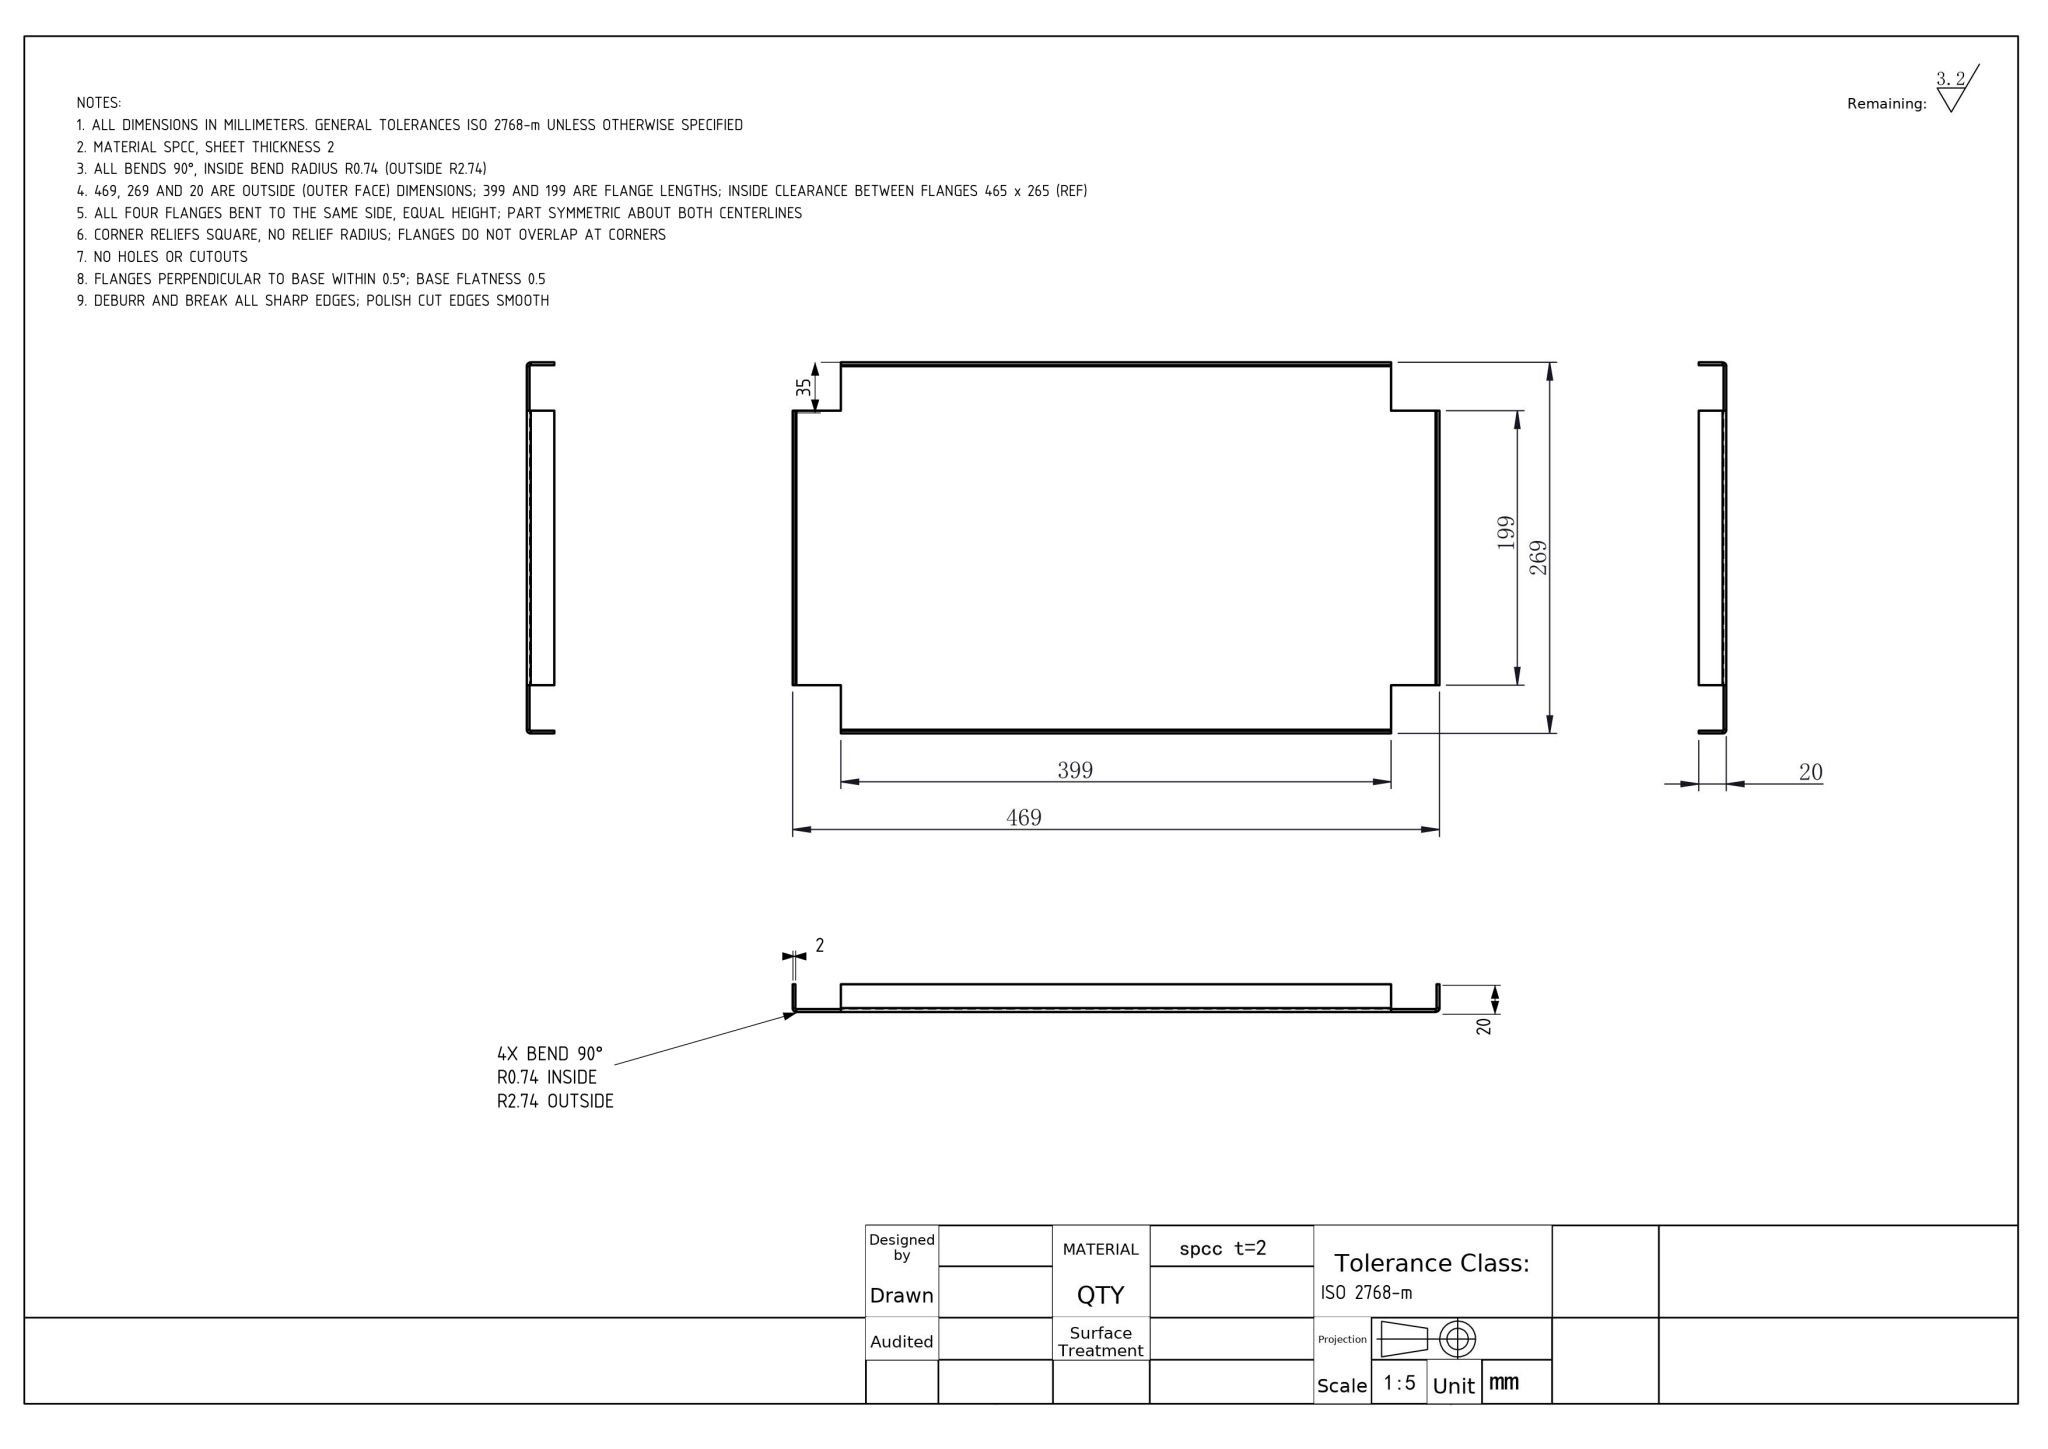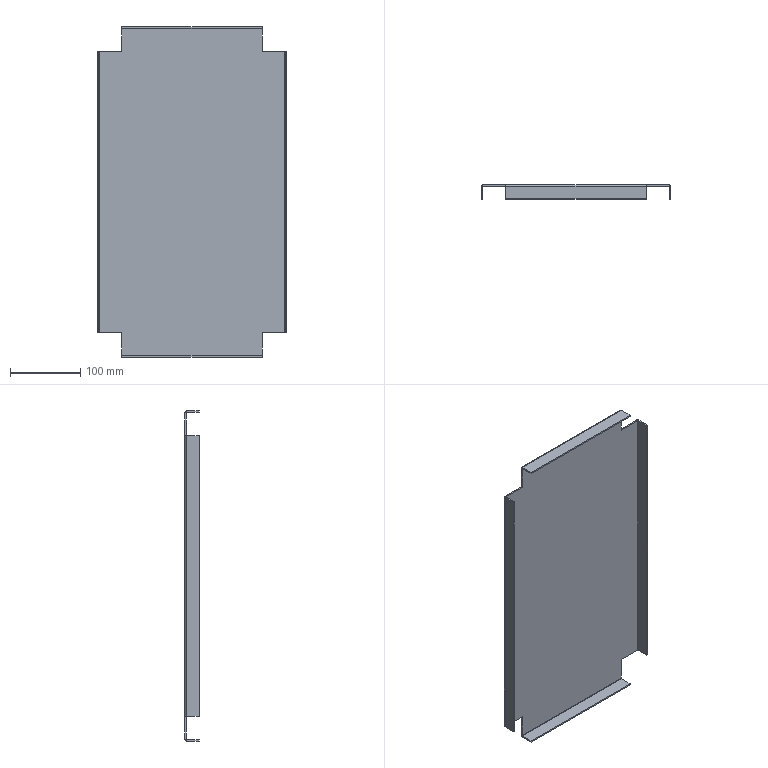Part | NX | mm | 1 solid | 46 faces | box 269 x 20 x 469 mm | volume 283795 mm3 | plane 38 | cylinder 8 | commonest cylinder face diameters 5.473 x4 1.473 x4